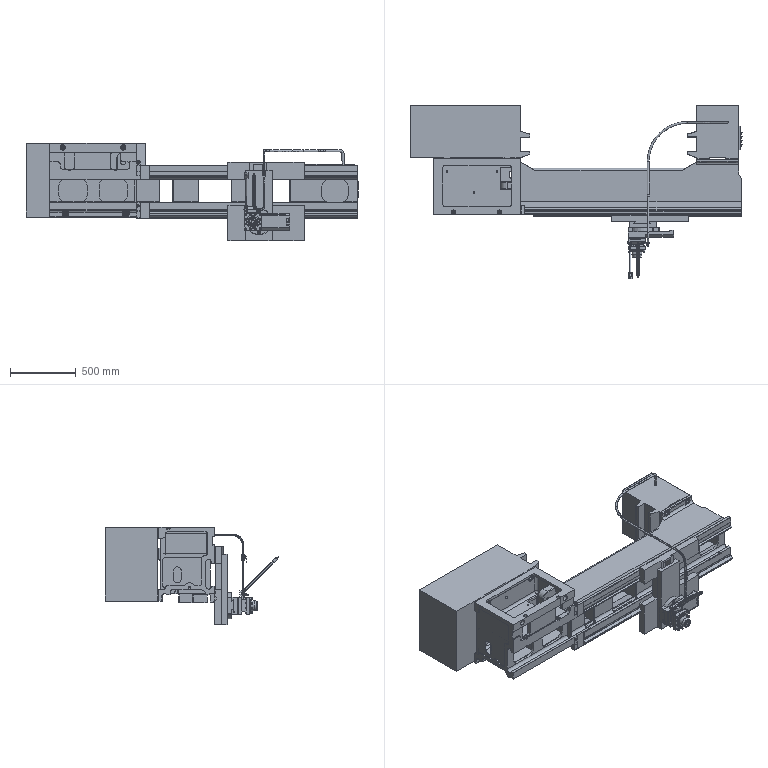Assembly | NX | mm | 38 component files | 72 solids | 2772 faces | box 2525 x 1322.1 x 738.98 mm | volume 291576106 mm3 | plane 1346 | cylinder 816 | cone 204 | spline 145 | torus 141 | sphere 79 | other 41 | commonest cylinder face diameters 10 x98 12 x82 40 x55 2 x53 0.86 x48 4 x46 1 x38 18 x38
Bill of materials:
unnamed part 1 | 1 |  | Square block with an H-shaped side profile. One large face has a pattern of round holes around its edge, a few smaller holes, and a shallow circular recess in the center.
unnamed part 2 | 1 |  | Plate made of a round disc merged with a wider rectangular bar. It has three round holes in a line, one square through-opening, two long grooves, and a dovetail-shaped tongue on one face.
unnamed part 3 | 1 |  | Long block whose end profile has a V-shaped notch on top and a narrower rectangular tongue underneath, giving a T-like base. It has counterbored holes on two faces, one cross hole, and a small stub sticking out of one end face.
unnamed part 4 | 1 |  | Thin rectangular plate with a dovetail-shaped groove along one short edge. Near the other end it has a small central through-hole surrounded by concentric shallow circular recesses, plus a small notch below the hole.
unnamed part 5 | 1 |  | Slender round rod bent into a three-dimensional frame shape, with several straight runs joined by curved bends. The ends are short hooks.
unnamed part 6 | 1 |  | Inline body that looks like a lever-operated valve. It has hex-shaped sections, a cylindrical central body, a flat bent lever handle with a domed knob at the pivot, a plain tube spigot at one end, and a ribbed (barbed) spigot at the other.
unnamed part 7 | 1 |  | Long beam-like housing with an open rectangular box pocket at one end. It has rectangular windows with rounded corners in the side walls, internal cross ribs, ledges running along its length, and a small flange tab with holes at the far end.
unnamed part 8 | 1 |  | Stepped shaft with two splined or knurled sections of different lengths, separated by a plain neck. Beyond them are a smooth, smaller-diameter shaft, a pair of thin ring collars, and a conical pointed tip.
unnamed part 9 | 1 |  | Flanged cup or cap: a circular flange with 8 holes in a ring, a cylindrical body that tapers to a rounded closed end, and concentric raised rings on the end face.
unnamed part 10 | 12 |  | Straight cylindrical pin with a square head at one end (the head's corners are rounded to the shank's outline). A thin collar sits between the head and the shank, and the far end is chamfered.
unnamed part 11 | 3 |  | Short fitting body: a hex section between a plain cylindrical spigot and a round collar end with a central bore. There is a groove or recessed ring between the hex and the collar.
unnamed part 12 | 1 |  | Long, thin round rod with a rectangular block head at one end. The head has a U-shaped slot, three small holes in a row, and a thin angled tab. The far end of the rod steps down to a smaller-diameter tip.
unnamed part 13 | 1 |  | Round cap-like body with a knurled outer surface. A conical top face narrows into a thin, hollow cylindrical stem.
unnamed part 14 | 1 |  | Rectangular box-shaped body. Its side faces have small tabs and small holes, one end has a notched/stepped profile, and one face has a group of four parallel slots.
unnamed part 15 | 6 |  | Fastener-like part: a cylindrical head with a hexagonal socket recess on a long, smooth cylindrical shank with a chamfered tip.
unnamed part 16 | 1 |  | Long, slender rod made of many repeated segments. Each segment has a cone-and-collar profile, with stepped flanged end fittings at both ends.
unnamed part 17 | 2 |  | Plain solid cylinder (pin-like) with chamfered edges at both ends.
unnamed part 18 | 1 |  | Flat plate with an H-like/stepped outline. Rectangular notches cut into the sides leave a central web, and there is a rectangular through-slot in the lower region. A narrow trapezoidal rib runs along one face.
unnamed part 19 | 1 |  | Elongated stepped block. A thicker square section at one end carries a cylindrical boss with a through-hole and two shallow circular recesses. The thinner extended section has chamfered edges, a raised lip at its end, an obround pad with a small hole, and a transverse hole near the end.
Mates:
1. fix | tool_holder_body 1 component
2. touch align | motor 1 | tool_holder_body 1
3. concentric | motor 1 | tool_holder_body 1
4. touch align | screw 12 | tool_holder_body 1
5. distance | screw 12 | tool_holder_body 1
6. concentric | 6_locating_pin 2 | motor 1
7. touch align | screw 4 | tool_holder_body 1
8. touch align | screw 5 | tool_holder_body 1
9. touch align | screw 6 | tool_holder_body 1
10. touch align | screw 7 | tool_holder_body 1
11. touch align | screw 8 | tool_holder_body 1
12. touch align | screw 9 | tool_holder_body 1
13. touch align | screw 10 | tool_holder_body 1
14. touch align | screw 11 | tool_holder_body 1
15. touch align | screw 3 | tool_holder_body 1
16. distance | screw 3 | tool_holder_body 1
17. distance | tool_holder_body 1 | screw 11
18. distance | screw 10 | tool_holder_body 1
19. distance | tool_holder_body 1 | screw 9
20. distance | screw 8 | tool_holder_body 1
21. distance | screw 7 | tool_holder_body 1
22. distance | tool_holder_body 1 | screw 6
23. distance | screw 5 | tool_holder_body 1
24. distance | screw 4 | tool_holder_body 1
25. touch align | screw 2 | tool_holder_body 1
26. touch align | screw 1 | tool_holder_body 1
27. distance | screw 1 | tool_holder_body 1
28. distance | tool_holder_body 1 | screw 2
29. concentric | M6x30_hex_screw 6 | motor 1
30. fix | assembly component
31. bond | M6x30_hex_screw 6 component | assembly component
32. bond | M6x30_hex_screw 5 component | assembly component
33. circular | assembly datumaxis | assembly cartesiancoordinatesystem | assembly cartesiancoordinatesystem | assembly cartesiancoordinatesystem | assembly cartesiancoordinatesystem | assembly cartesiancoordinatesystem | assembly cartesiancoordinatesystem
34. bond | M6x30_hex_screw 4 component | assembly component
35. bond | M6x30_hex_screw 3 component | assembly component
36. bond | M6x30_hex_screw 2 component | assembly component
37. bond | M6x30_hex_screw 1 component | assembly component
38. concentric | 6_locating_pin 1 | motor 1
39. touch align | valve 1 | assembly line
40. parallel | valve 1 | assembly datumplane
41. concentric | air_pipe_connector 1 | assembly edge
42. concentric | air_pipe_connector 3 | assembly edge
43. concentric | air_pipe_connector 2 | assembly edge
44. concentric | universal_joint_tube 1 | air_pipe_connector 3
45. concentric | model1 1 | air_pipe_connector 2
46. parallel | model1 1 | assembly face
47. concentric | universal_joint_tube 1 | nozzle 1
48. touch align | adjustment_knob 1 | assembly face
49. distance | adjustment_knob 1 | assembly face
50. fix | lathe_base 1 component
51. touch align | lathe_bed 1 face | lathe_base 1 face
52. concentric | lathe_base 1 edge | lathe_bed 1 edge
53. parallel | lathe_bed 1 face | lathe_base 1 face
54. parallel | large_base 1 face | lathe_bed 1 face
55. touch align | large_base 1 face | lathe_bed 1 face
56. touch align | large_base 1 face | lathe_bed 1 face
57. touch align | dovetail_seat 1 face | large_base 1 face
58. touch align | tool_holder_base 1 face | dovetail_seat 1 face
59. touch align | tool_holder_base 1 face | dovetail_seat 1 face
60. parallel | tool_holder_base 1 face | lathe_bed 1 face
61. touch align | tool_holder_dovetail_base 1 face | tool_holder_base 1 face
62. touch align | tool_holder_dovetail_base 1 face | tool_holder_base 1 face
63. touch align | tool_holder_dovetail_base 1 face | tool_holder_base 1 face
64. touch align | tool_holder_assy 1 face | tool_holder_dovetail_base 1 face
65. touch align | tool_holder_assy 1 face | tool_holder_dovetail_base 1 face
66. parallel | water_pipe 1 face | tool_holder_dovetail_base 1 face
67. fix | water_pipe 1 component
68. distance | magnetic_base 1 face | tool_holder_assy 1 face
69. touch align | dovetail_seat 1 face | large_base 1 face
70. touch align | dovetail_seat 1 face | large_base 1 face
71. touch align | magnetic_base 1 face | tool_holder_assy 1 face
72. fix | magnetic_base 1 component